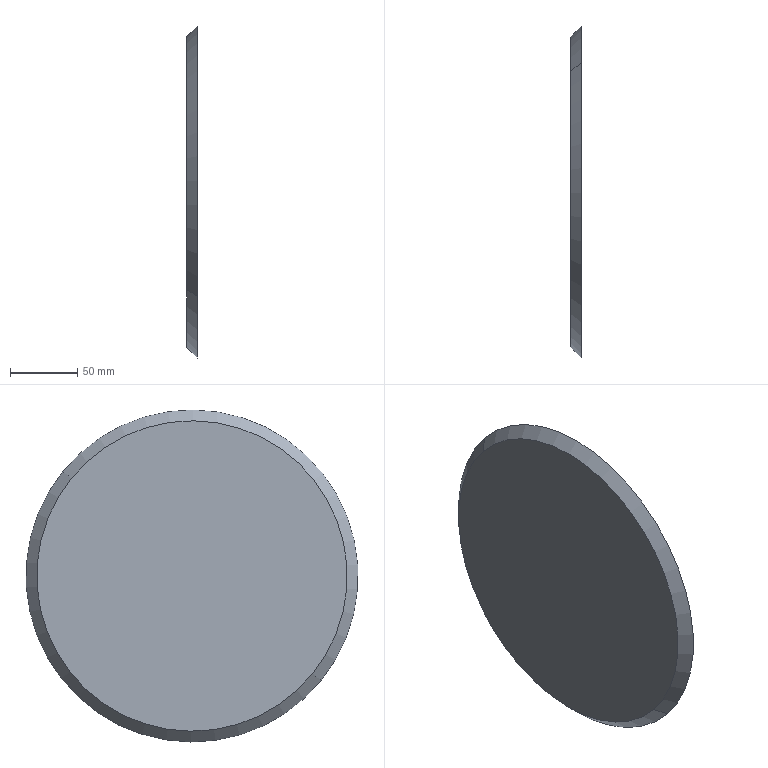Component | SolidWorks | BrakeShoe-1 | 1 solid | 4 faces | box 8 x 246 x 246 mm | volume 356039 mm3 | cone 2 | plane 2
build123d program:
from build123d import *


with BuildPart() as part:
    # Sketch2 → Revolve1 (revolve)
    with BuildSketch(Plane.XY):
        Polygon((0, 0), (0, 115), (8, 123), (8, 0), align=None)
    revolve(axis=Axis((8, 0, 0), (-1, 0, 0)))


solid = part.part

# Placed as in the assembly
solid = solid.moved(Location((-261.5, 0, 0), (0, 0, 0)))
STEP:
#1=COLOUR_RGB('',0.7922,0.8196,0.9333);
#2=FILL_AREA_STYLE_COLOUR('',#1);
#3=FILL_AREA_STYLE('',(#2));
#4=SURFACE_STYLE_FILL_AREA(#3);
#5=SURFACE_SIDE_STYLE('',(#4));
#6=SURFACE_STYLE_USAGE(.BOTH.,#5);
#7=PRESENTATION_STYLE_ASSIGNMENT((#6));
#8=CARTESIAN_POINT('',(-10.295,3.52,2.847));
#9=VERTEX_POINT('',#8);
#10=CARTESIAN_POINT('',(-10.295,-3.52,-2.847));
#11=VERTEX_POINT('',#10);
#12=CARTESIAN_POINT('',(-10.295,0.,-0.));
#13=DIRECTION('',(1.,0.,-0.));
#14=DIRECTION('',(0.,0.7775,0.6288));
#15=AXIS2_PLACEMENT_3D('',#12,#13,#14);
#16=CIRCLE('',#15,4.528);
#17=EDGE_CURVE('',#9,#11,#16,.T.);
#18=ORIENTED_EDGE('',*,*,#17,.T.);
#19=CARTESIAN_POINT('',(-9.98,-3.765,-3.045));
#20=VERTEX_POINT('',#19);
#21=CARTESIAN_POINT('',(-9.98,-3.765,-3.045));
#22=DIRECTION('',(0.7071,-0.5498,-0.4447));
#23=VECTOR('',#22,39.37);
#24=LINE('',#21,#23);
#25=EDGE_CURVE('',#11,#20,#24,.T.);
#26=ORIENTED_EDGE('',*,*,#25,.T.);
#27=CARTESIAN_POINT('',(-9.98,3.765,3.045));
#28=VERTEX_POINT('',#27);
#29=CARTESIAN_POINT('',(-9.98,0.,-0.));
#30=DIRECTION('',(1.,0.,-0.));
#31=DIRECTION('',(0.,0.7775,0.6288));
#32=AXIS2_PLACEMENT_3D('',#29,#30,#31);
#33=CIRCLE('',#32,4.843);
#34=EDGE_CURVE('',#28,#20,#33,.T.);
#35=ORIENTED_EDGE('',*,*,#34,.F.);
#36=CARTESIAN_POINT('',(-9.98,3.765,3.045));
#37=DIRECTION('',(0.7071,0.5498,0.4447));
#38=VECTOR('',#37,39.37);
#39=LINE('',#36,#38);
#40=EDGE_CURVE('',#9,#28,#39,.T.);
#41=ORIENTED_EDGE('',*,*,#40,.F.);
#42=EDGE_LOOP('',(#18,#26,#35,#41));
#43=FACE_OUTER_BOUND('',#42,.T.);
#44=CARTESIAN_POINT('',(-9.98,0.,-0.));
#45=DIRECTION('',(1.,0.,-0.));
#46=DIRECTION('',(0.,0.7775,0.6288));
#47=AXIS2_PLACEMENT_3D('',#44,#45,#46);
#48=CONICAL_SURFACE('',#47,4.843,0.7854);
#49=ADVANCED_FACE('',(#43),#48,.T.);
#50=ORIENTED_EDGE('',*,*,#17,.F.);
#51=CARTESIAN_POINT('',(-10.295,0.,-0.));
#52=DIRECTION('',(1.,0.,-0.));
#53=DIRECTION('',(0.,0.7775,0.6288));
#54=AXIS2_PLACEMENT_3D('',#51,#52,#53);
#55=CIRCLE('',#54,4.528);
#56=EDGE_CURVE('',#11,#9,#55,.T.);
#57=ORIENTED_EDGE('',*,*,#56,.F.);
#58=EDGE_LOOP('',(#50,#57));
#59=FACE_OUTER_BOUND('',#58,.T.);
#60=CARTESIAN_POINT('',(-10.295,0.,-0.));
#61=DIRECTION('',(-1.,-0.,0.));
#62=DIRECTION('',(0.,-0.7775,-0.6288));
#63=AXIS2_PLACEMENT_3D('',#60,#61,#62);
#64=PLANE('',#63);
#65=ADVANCED_FACE('',(#59),#64,.T.);
#66=ORIENTED_EDGE('',*,*,#25,.F.);
#67=ORIENTED_EDGE('',*,*,#56,.T.);
#68=ORIENTED_EDGE('',*,*,#40,.T.);
#69=CARTESIAN_POINT('',(-9.98,0.,-0.));
#70=DIRECTION('',(1.,0.,-0.));
#71=DIRECTION('',(0.,0.7775,0.6288));
#72=AXIS2_PLACEMENT_3D('',#69,#70,#71);
#73=CIRCLE('',#72,4.843);
#74=EDGE_CURVE('',#20,#28,#73,.T.);
#75=ORIENTED_EDGE('',*,*,#74,.F.);
#76=EDGE_LOOP('',(#66,#67,#68,#75));
#77=FACE_OUTER_BOUND('',#76,.T.);
#78=CARTESIAN_POINT('',(-9.98,0.,-0.));
#79=DIRECTION('',(1.,0.,-0.));
#80=DIRECTION('',(0.,0.7775,0.6288));
#81=AXIS2_PLACEMENT_3D('',#78,#79,#80);
#82=CONICAL_SURFACE('',#81,4.843,0.7854);
#83=ADVANCED_FACE('',(#77),#82,.T.);
#84=ORIENTED_EDGE('',*,*,#34,.T.);
#85=ORIENTED_EDGE('',*,*,#74,.T.);
#86=EDGE_LOOP('',(#84,#85));
#87=FACE_OUTER_BOUND('',#86,.T.);
#88=CARTESIAN_POINT('',(-9.98,3.765,3.045));
#89=DIRECTION('',(1.,0.,-0.));
#90=DIRECTION('',(-0.,0.7775,0.6288));
#91=AXIS2_PLACEMENT_3D('',#88,#89,#90);
#92=PLANE('',#91);
#93=ADVANCED_FACE('',(#87),#92,.T.);
#94=CLOSED_SHELL('',(#49,#65,#83,#93));
#95=MANIFOLD_SOLID_BREP('',#94);
#96=STYLED_ITEM('',(#7),#95);
#97=PRESENTATION_LAYER_ASSIGNMENT('','',(#96));
#98=CARTESIAN_POINT('',(0.,0.,0.));
#99=DIRECTION('',(0.,0.,1.));
#100=DIRECTION('',(1.,0.,0.));
#101=AXIS2_PLACEMENT_3D('',#98,#99,#100);
#102=(LENGTH_UNIT()NAMED_UNIT(*)SI_UNIT($,.METRE.));
#103=LENGTH_MEASURE_WITH_UNIT(LENGTH_MEASURE(0.0254),#102);
#104=DIMENSIONAL_EXPONENTS(1.,0.,0.,0.,0.,0.,0.);
#105=(CONVERSION_BASED_UNIT('',#103)LENGTH_UNIT()NAMED_UNIT(#104));
#106=UNCERTAINTY_MEASURE_WITH_UNIT(LENGTH_MEASURE(0.00001),#105,'','');
#107=(NAMED_UNIT(*)PLANE_ANGLE_UNIT()SI_UNIT($,.RADIAN.));
#108=(NAMED_UNIT(*)SI_UNIT($,.STERADIAN.)SOLID_ANGLE_UNIT());
#109=(GEOMETRIC_REPRESENTATION_CONTEXT(3)GLOBAL_UNCERTAINTY_ASSIGNED_CONTEXT((#106))GLOBAL_UNIT_ASSIGNED_CONTEXT((#105,#107,#108))REPRESENTATION_CONTEXT('',''));
#110=ADVANCED_BREP_SHAPE_REPRESENTATION('',(#95,#101),#109);
#111=(LENGTH_UNIT()NAMED_UNIT(*)SI_UNIT($,.METRE.));
#112=LENGTH_MEASURE_WITH_UNIT(LENGTH_MEASURE(0.0254),#111);
#113=DIMENSIONAL_EXPONENTS(1.,0.,0.,0.,0.,0.,0.);
#114=(CONVERSION_BASED_UNIT('',#112)LENGTH_UNIT()NAMED_UNIT(#113));
#115=UNCERTAINTY_MEASURE_WITH_UNIT(LENGTH_MEASURE(0.00001),#114,'','');
#116=(NAMED_UNIT(*)PLANE_ANGLE_UNIT()SI_UNIT($,.RADIAN.));
#117=(NAMED_UNIT(*)SI_UNIT($,.STERADIAN.)SOLID_ANGLE_UNIT());
#118=(GEOMETRIC_REPRESENTATION_CONTEXT(3)GLOBAL_UNCERTAINTY_ASSIGNED_CONTEXT((#115))GLOBAL_UNIT_ASSIGNED_CONTEXT((#114,#116,#117))REPRESENTATION_CONTEXT('',''));
#119=MECHANICAL_DESIGN_GEOMETRIC_PRESENTATION_REPRESENTATION('',(#96),#118);